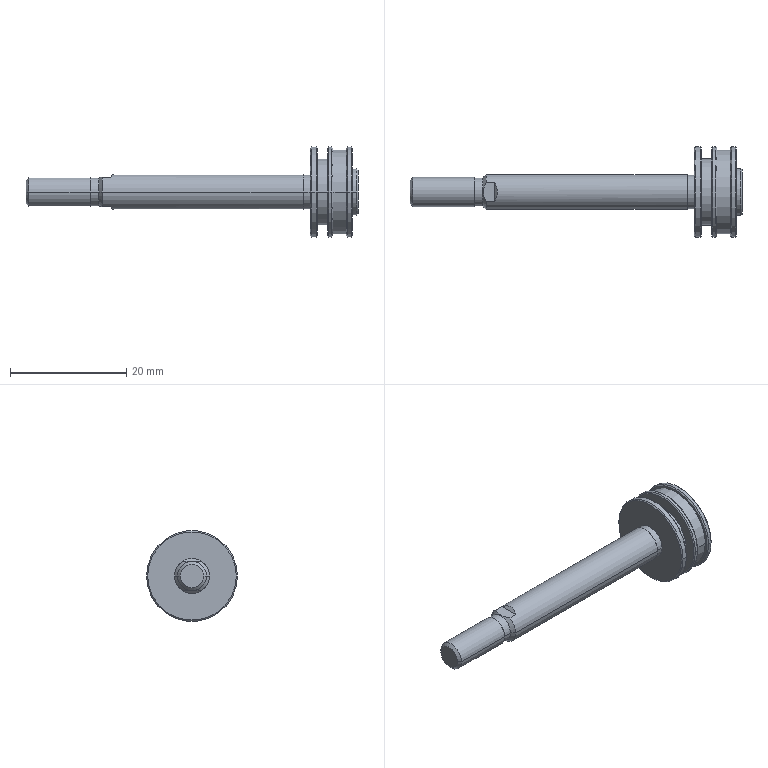Component | SolidWorks | 09MD-16x10-S (0)-1_09MD 16x10-S10 - Rod-1 | 1 solid | 52 faces | box 57 x 15.6 x 15.6 mm | volume 2453 mm3 | cylinder 20 | cone 18 | plane 14 | commonest cylinder face diameters 15.6 x6 8 x2 14.4 x2 11.4 x2 5.8 x2 6 x2 4.8 x2 5 x2
build123d program:
from build123d import *

# Parameters (mm, degrees)
CUT_EXTRUDE1_DEPTH      = 6
CUT_EXTRUDE1_DEPTH_BACK = 6


with BuildPart() as part:
    # Sketch1 → Revolve1 (revolve)
    with BuildSketch(Plane.XY, mode=Mode.PRIVATE) as revolve1_sk:
        Polygon((-16, 0), (-16, 2.01), (-15.509, 2.5), (-5, 2.5), (-5, 2.4), (-3.5, 2.4), (-2.9, 3), (31.6, 3), (31.6, 2.9), (32.8, 2.9), (32.8, 7.6), (33, 7.8), (33.8, 7.8), (34, 7.6), (34, 5.7), (35.8, 5.7), (35.8, 7.6), (36, 7.8), (36.5, 7.8), (36.7, 7.6), (36.7, 7.2), (39, 7.2), (39, 7.6), (39.2, 7.8), (39.8, 7.8), (40, 7.6), (40, 4), (40.8, 4), (41, 3.8), (41, 0), align=None)
    revolve(revolve1_sk.sketch.rotate(Axis((41, 0, 0), (-1, 0, 0)), 270), axis=Axis((41, 0, 0), (-1, 0, 0)))

    # Sketch2 → Cut-Extrude1 (cut, two sides: drawn at the far end of the back side and taken through both)
    with BuildSketch(Plane.XY.offset(-CUT_EXTRUDE1_DEPTH_BACK)):
        Polygon((-19.5, 3), (-19.5, -3), (-1, -3), (-1.5, -2.5), (-18.5, -2.5), (-18.5, 2.5), (-1.5, 2.5), (-1, 3), align=None)
    extrude(amount=CUT_EXTRUDE1_DEPTH + CUT_EXTRUDE1_DEPTH_BACK, mode=Mode.SUBTRACT)


solid = part.part

# Placed as in the assembly
solid = solid.moved(Location((-640.359, -286.383, -30.256), (90, 0, 0)))